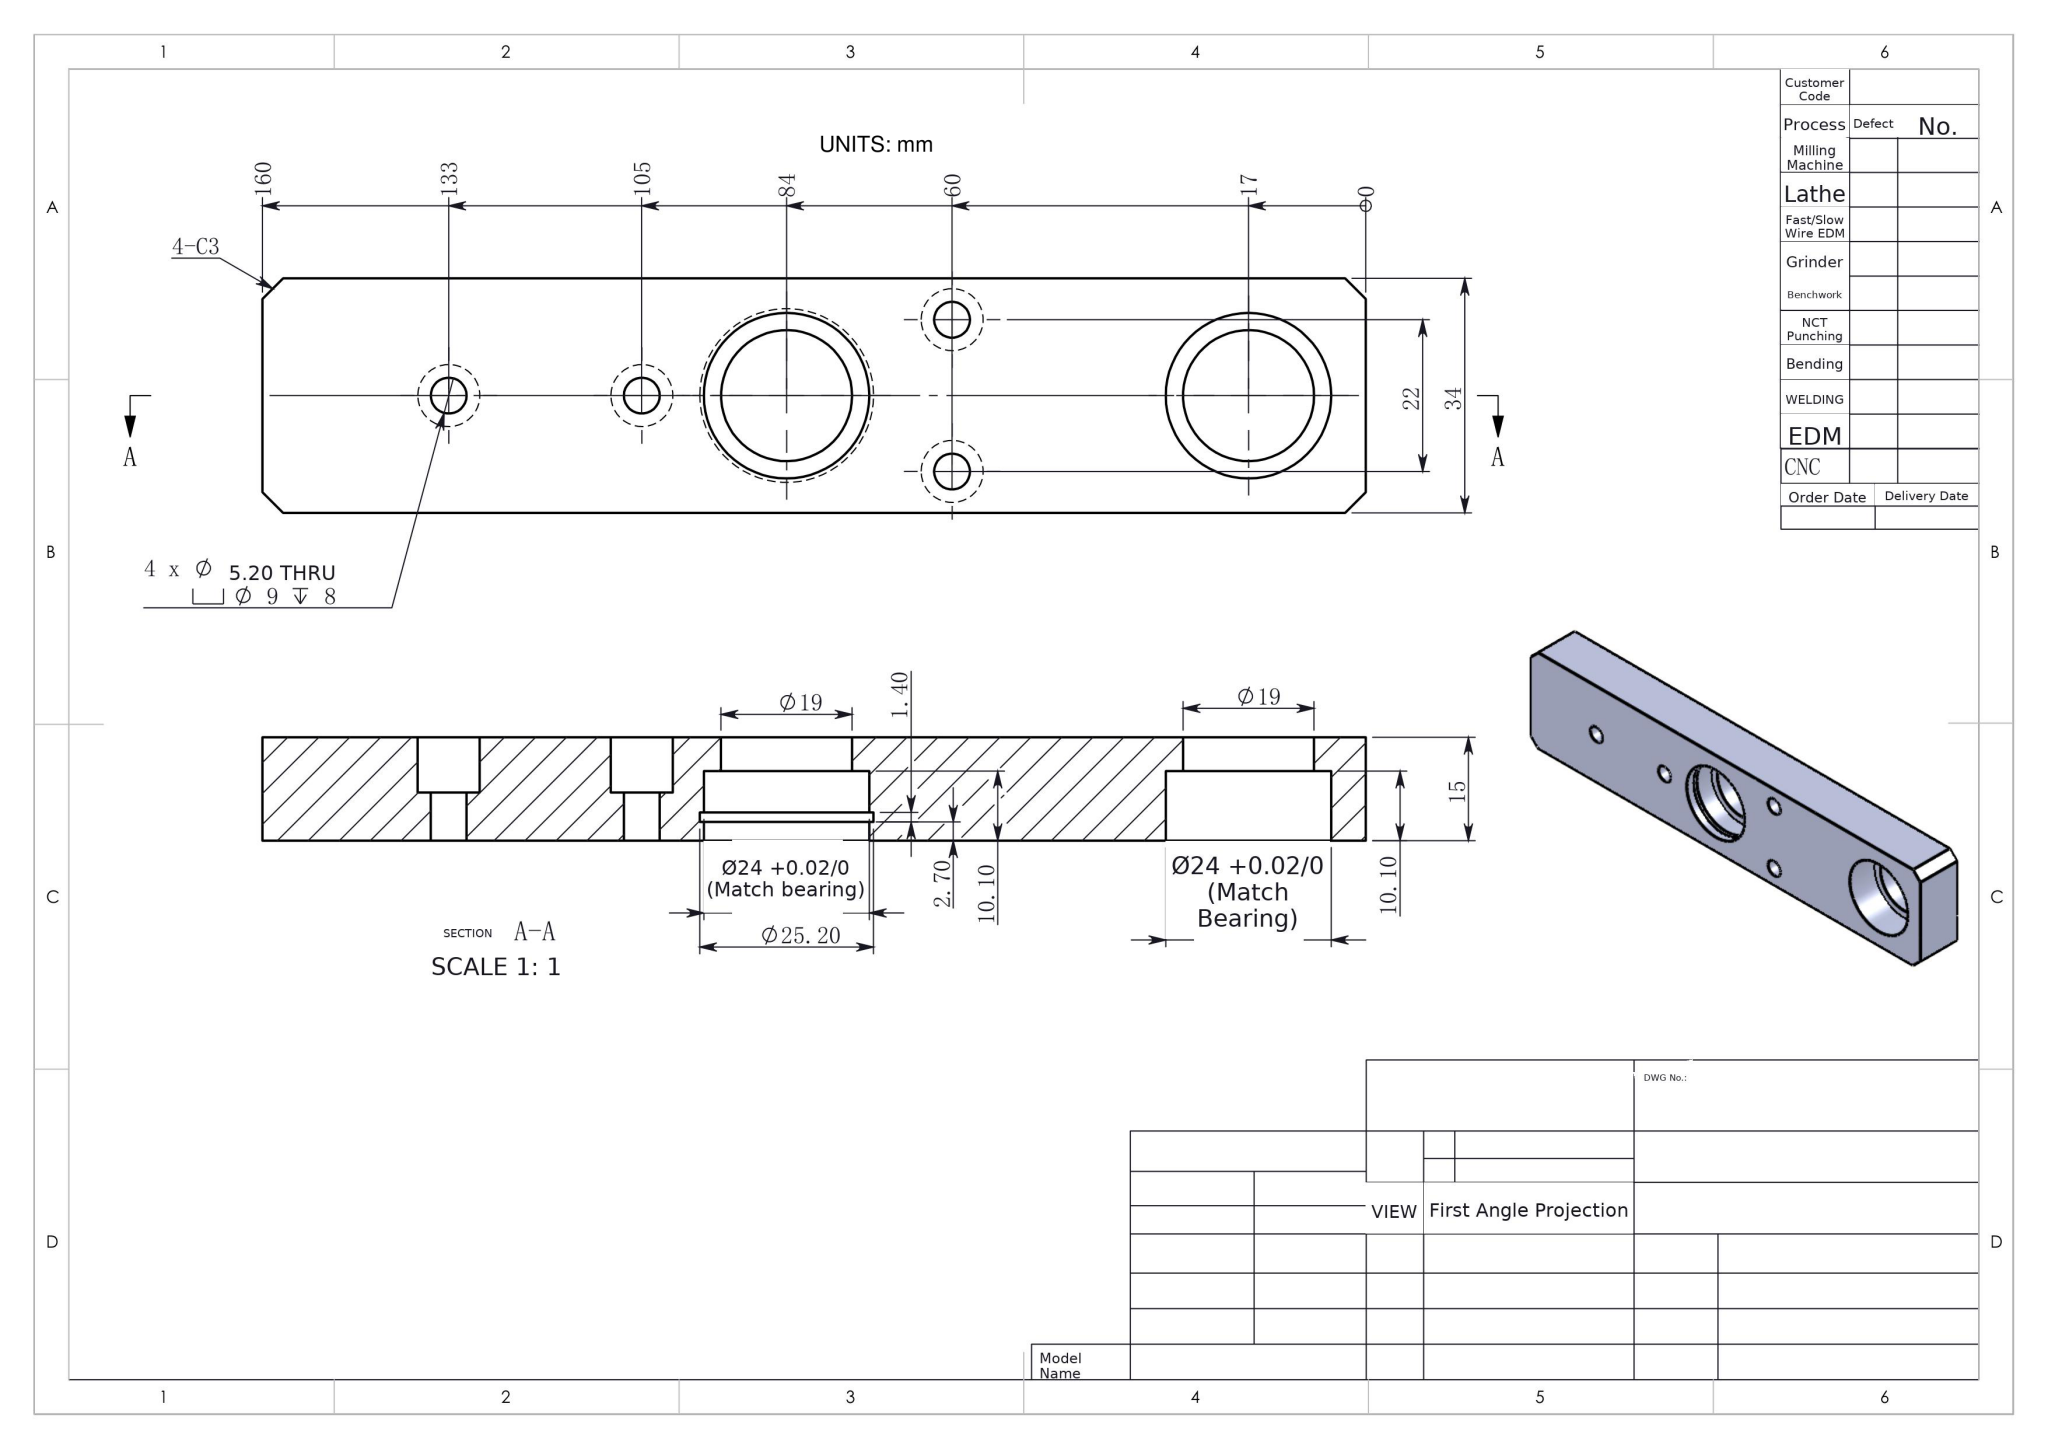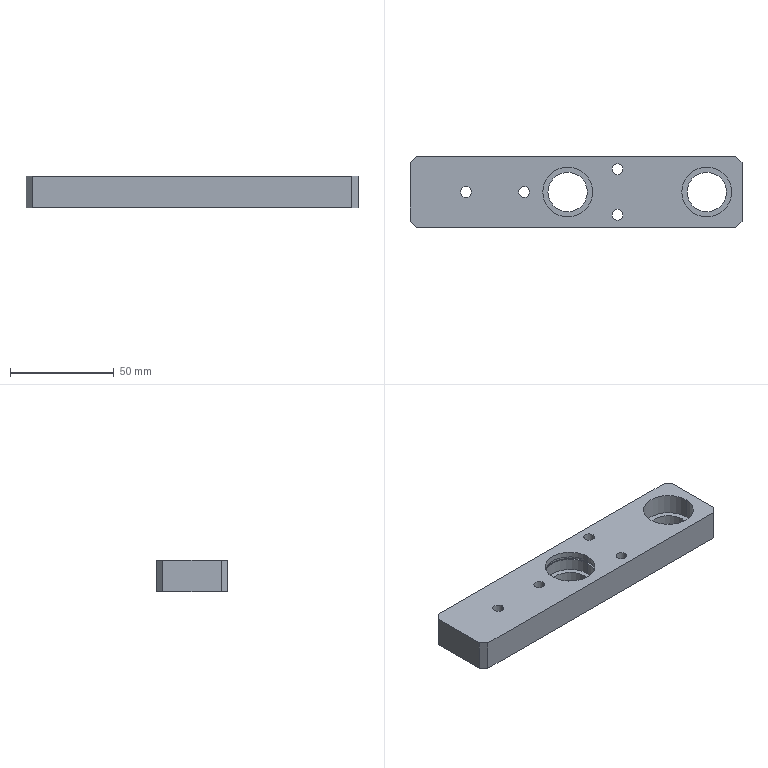Part | NX | mm | 1 solid | 46 faces | box 160 x 34 x 15 mm | volume 66718 mm3 | cylinder 28 | plane 18 | commonest cylinder face diameters 9 x8 5.2 x8 24 x6 19 x4 25.2 x2